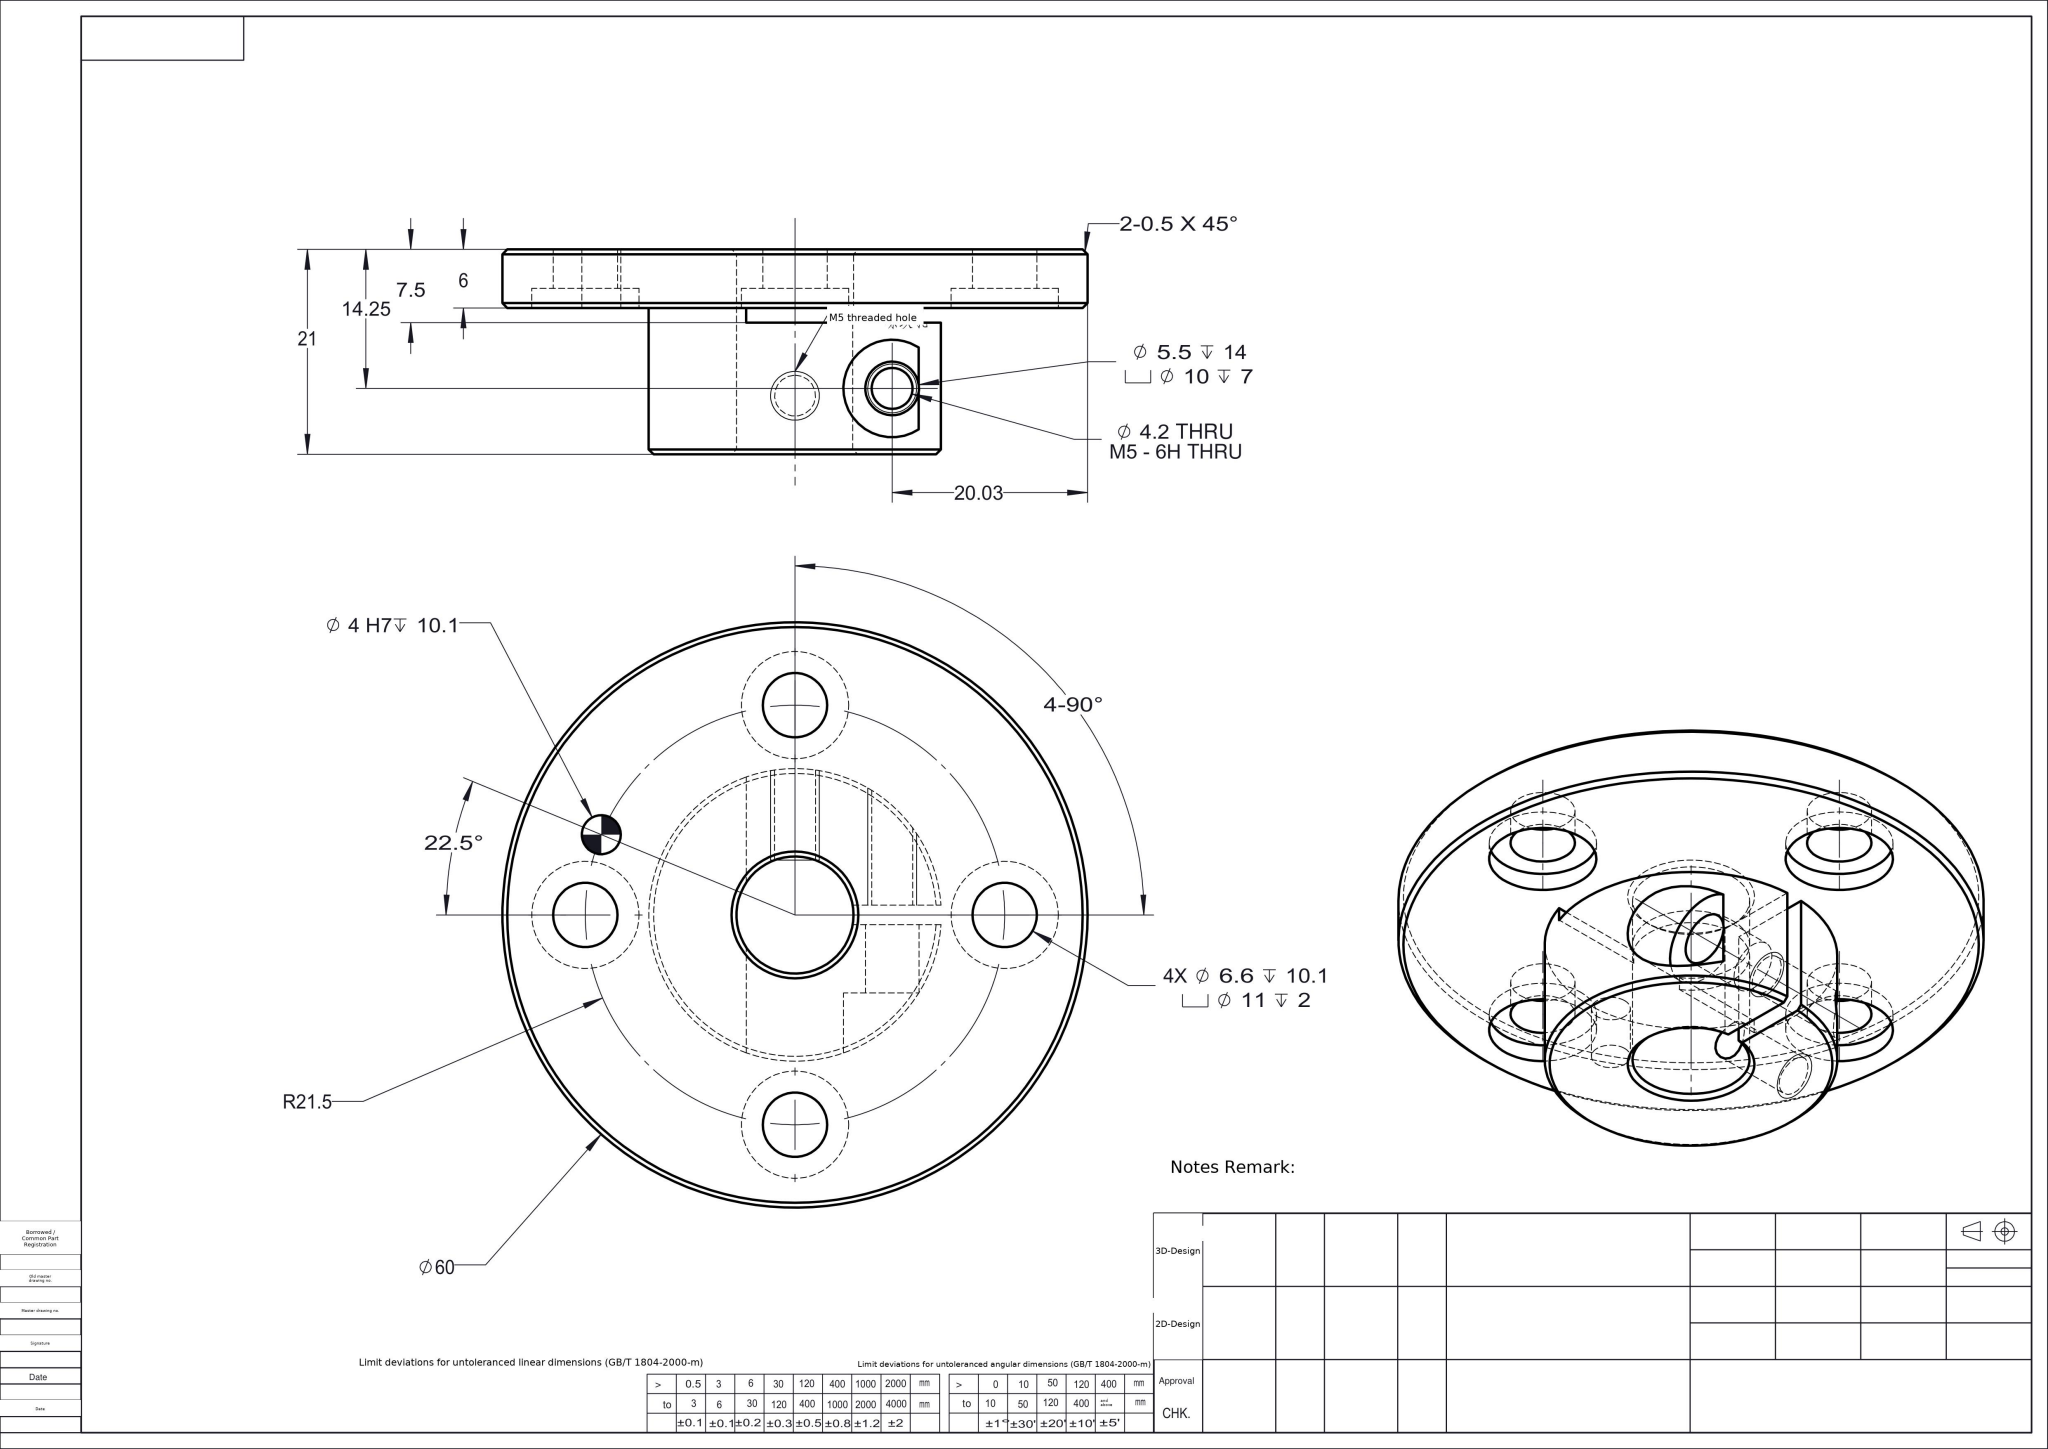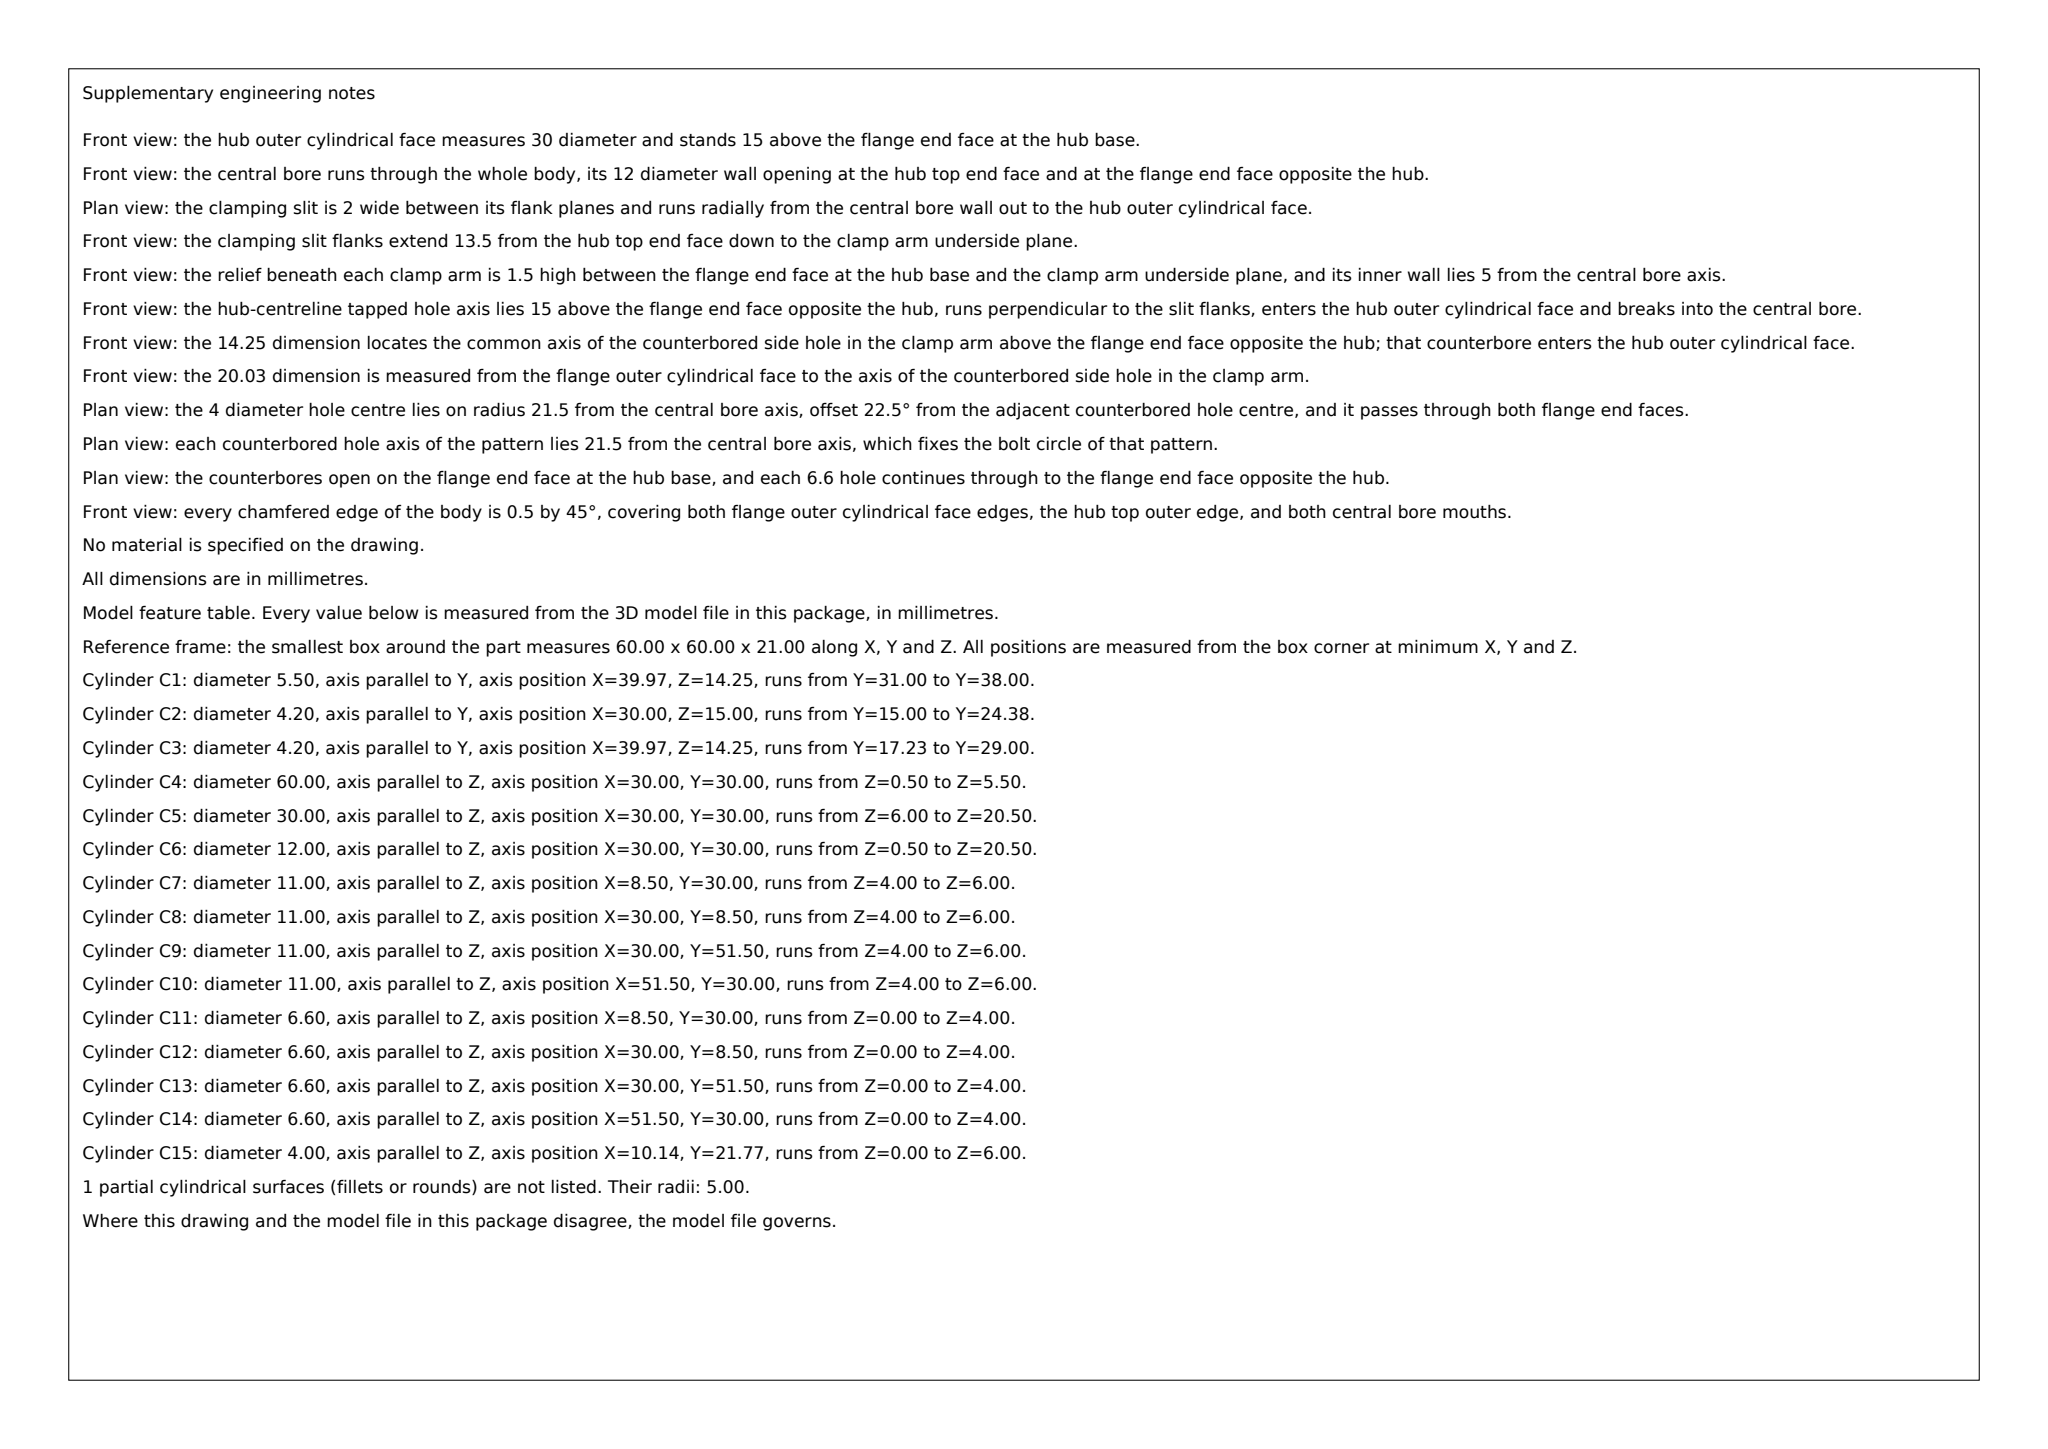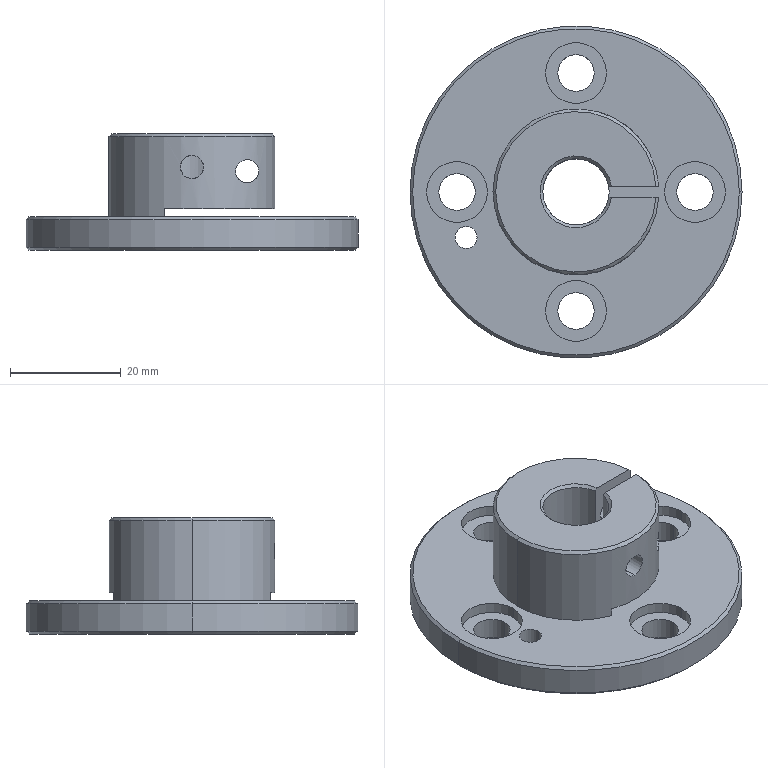Part | SolidWorks | mm | 1 solid | 56 faces | box 60 x 60 x 21 mm | volume 22247 mm3 | cylinder 33 | plane 14 | cone 9 | commonest cylinder face diameters 11 x8 6.6 x8 4.2 x4 10 x3 4 x2 5.5 x2 12 x2 30 x2
Drawing notes:
CENTRAL BORE Ø12 THRU, COAXIAL WITH Ø60 DISC (ON DISC AXIS), 0.5x45° CHAMFER BOTH ENDS | from the solid: cylinder dia 12.0 axis z at pos [30.0,30.0] length 20.0 + cones 90° ref dia 13.0 (x2); bbox z = 21.0
DISC (FLANGE) THICKNESS 6 - FROM BOTTOM FACE z=0 TO BOSS-SIDE FACE z=6 (Ø60 LAND 5 PLUS CHAMFER EACH FACE) | from the solid: axis_planes z=0.0 and z=6.0; cylinder dia 60.0 axis z length 5.0
CENTRAL BOSS Ø30 x 15 HIGH, COAXIAL WITH DISC AXIS, RISING FROM DISC FACE z=6 TO z=21; TOP EDGE 0.5x45° CHAMFER | from the solid: cylinder dia 30.0 axis z at pos [30.0,30.0] length 14.5; cone 90° ref dia 29.0; bbox z 21.0
M5 TAPPED HOLE (Ø4.2 TAP DRILL) IN BOSS: AXIS PARALLEL TO Y, ON DISC CENTRELINE x=30, 15 ABOVE DISC BOTTOM FACE, 9.38 DEEP | from the solid: cylinder dia 4.2 axis y pos [30.0,null,15.0] length 9.38
Ø5.5 / CBORE Ø10 COUNTERBORED HOLE: AXIS PARALLEL TO Y, 9.97 OFF DISC AXIS (x=39.97, = 20.03 FROM Ø60 EDGE) AND 14.25 ABOVE DISC BOTTOM FACE | from the solid: cylinders dia 5.5 and dia 10.0 axis y at pos [39.97,null,14.25]
CUT IN Ø30 BOSS (NOT A PLAIN CYLINDER): FLAT FACES NORMAL TO X AT x=25 (2 PLACES) AND A 2 WIDE SLOT BOUNDED BY FACES NORMAL TO Y AT y=29 AND y=31, PLUS FACE NORMAL TO Y AT y=38; COORDINATES FROM Ø60 DISC BBOX MIN CORNER (DISC AXIS x=30, y=30), CUT RUNS FROM FLOOR z=7.5 UP TO BOSS TOP z=21 | from the solid: axis_planes: ["z",7.5]:2 (cut floor) and ["z",21.0]:1 (boss top); ["x",25.0]:2, ["y",29.0]:1, ["y",31.0]:1, ["y",38.0]:1 - no cut face at z=6 other than the disc top face
Ø4.2 CROSS HOLE COAXIAL WITH THE Ø5.5 HOLE: AXIS PARALLEL TO Y AT x=39.97, 14.25 ABOVE DISC BOTTOM FACE; LENGTHS 10.21 AND 11.77 (ONE EACH SIDE) CONTINUING INBOARD BEYOND THE Ø5.5 BORE - SEPARATE FROM THE M5 HOLE OF NOTE 5 AT x=30 | from the solid: cylinders: 4.2 dia, y axis, pos (39.97, z=14.25), lengths 10.21 (1) and 11.77 (1)
Ø5.5 BORE AT x=39.97, z=14.25, AXIS PARALLEL TO Y: 7 LONG EACH SIDE (2 PLACES); Ø10 COUNTERBORE APPLIED BOTH SIDES - 3.21 DEEP (2 PLACES) AND 6.15 DEEP (1 PLACE) | from the solid: cylinders: 5.5 dia y axis at (39.97, z=14.25) length 7 (2); 10.0 dia y axis same position lengths 3.21 (2) and 6.15 (1)
BOSS CUT SIDE WALLS: 2 FLAT FACES NORMAL TO X AT x=25 (5 FROM DISC AXIS x=30, TOWARD -X SIDE); NO FACE AT x=35 EXISTS IN THE MODEL | from the solid: axis_planes [normal x, offset 25.0] count 2; no x=35 plane listed
BOSS CUT END WALL: FLAT FACE NORMAL TO Y AT y=38 (8 FROM DISC AXIS y=30) | from the solid: axis_planes [normal y, offset 38.0] count 1
BOSS CUT FLOOR: 2 HORIZONTAL FACES AT z=7.5 (7.5 ABOVE DISC BOTTOM FACE z=0, 1.5 ABOVE DISC TOP FACE z=6); CUT WALLS RUN FROM THIS FLOOR UP TO BOSS TOP z=21 | from the solid: axis_planes [normal z, offset 7.5] count 2; axis_planes z=6.0 and z=21.0